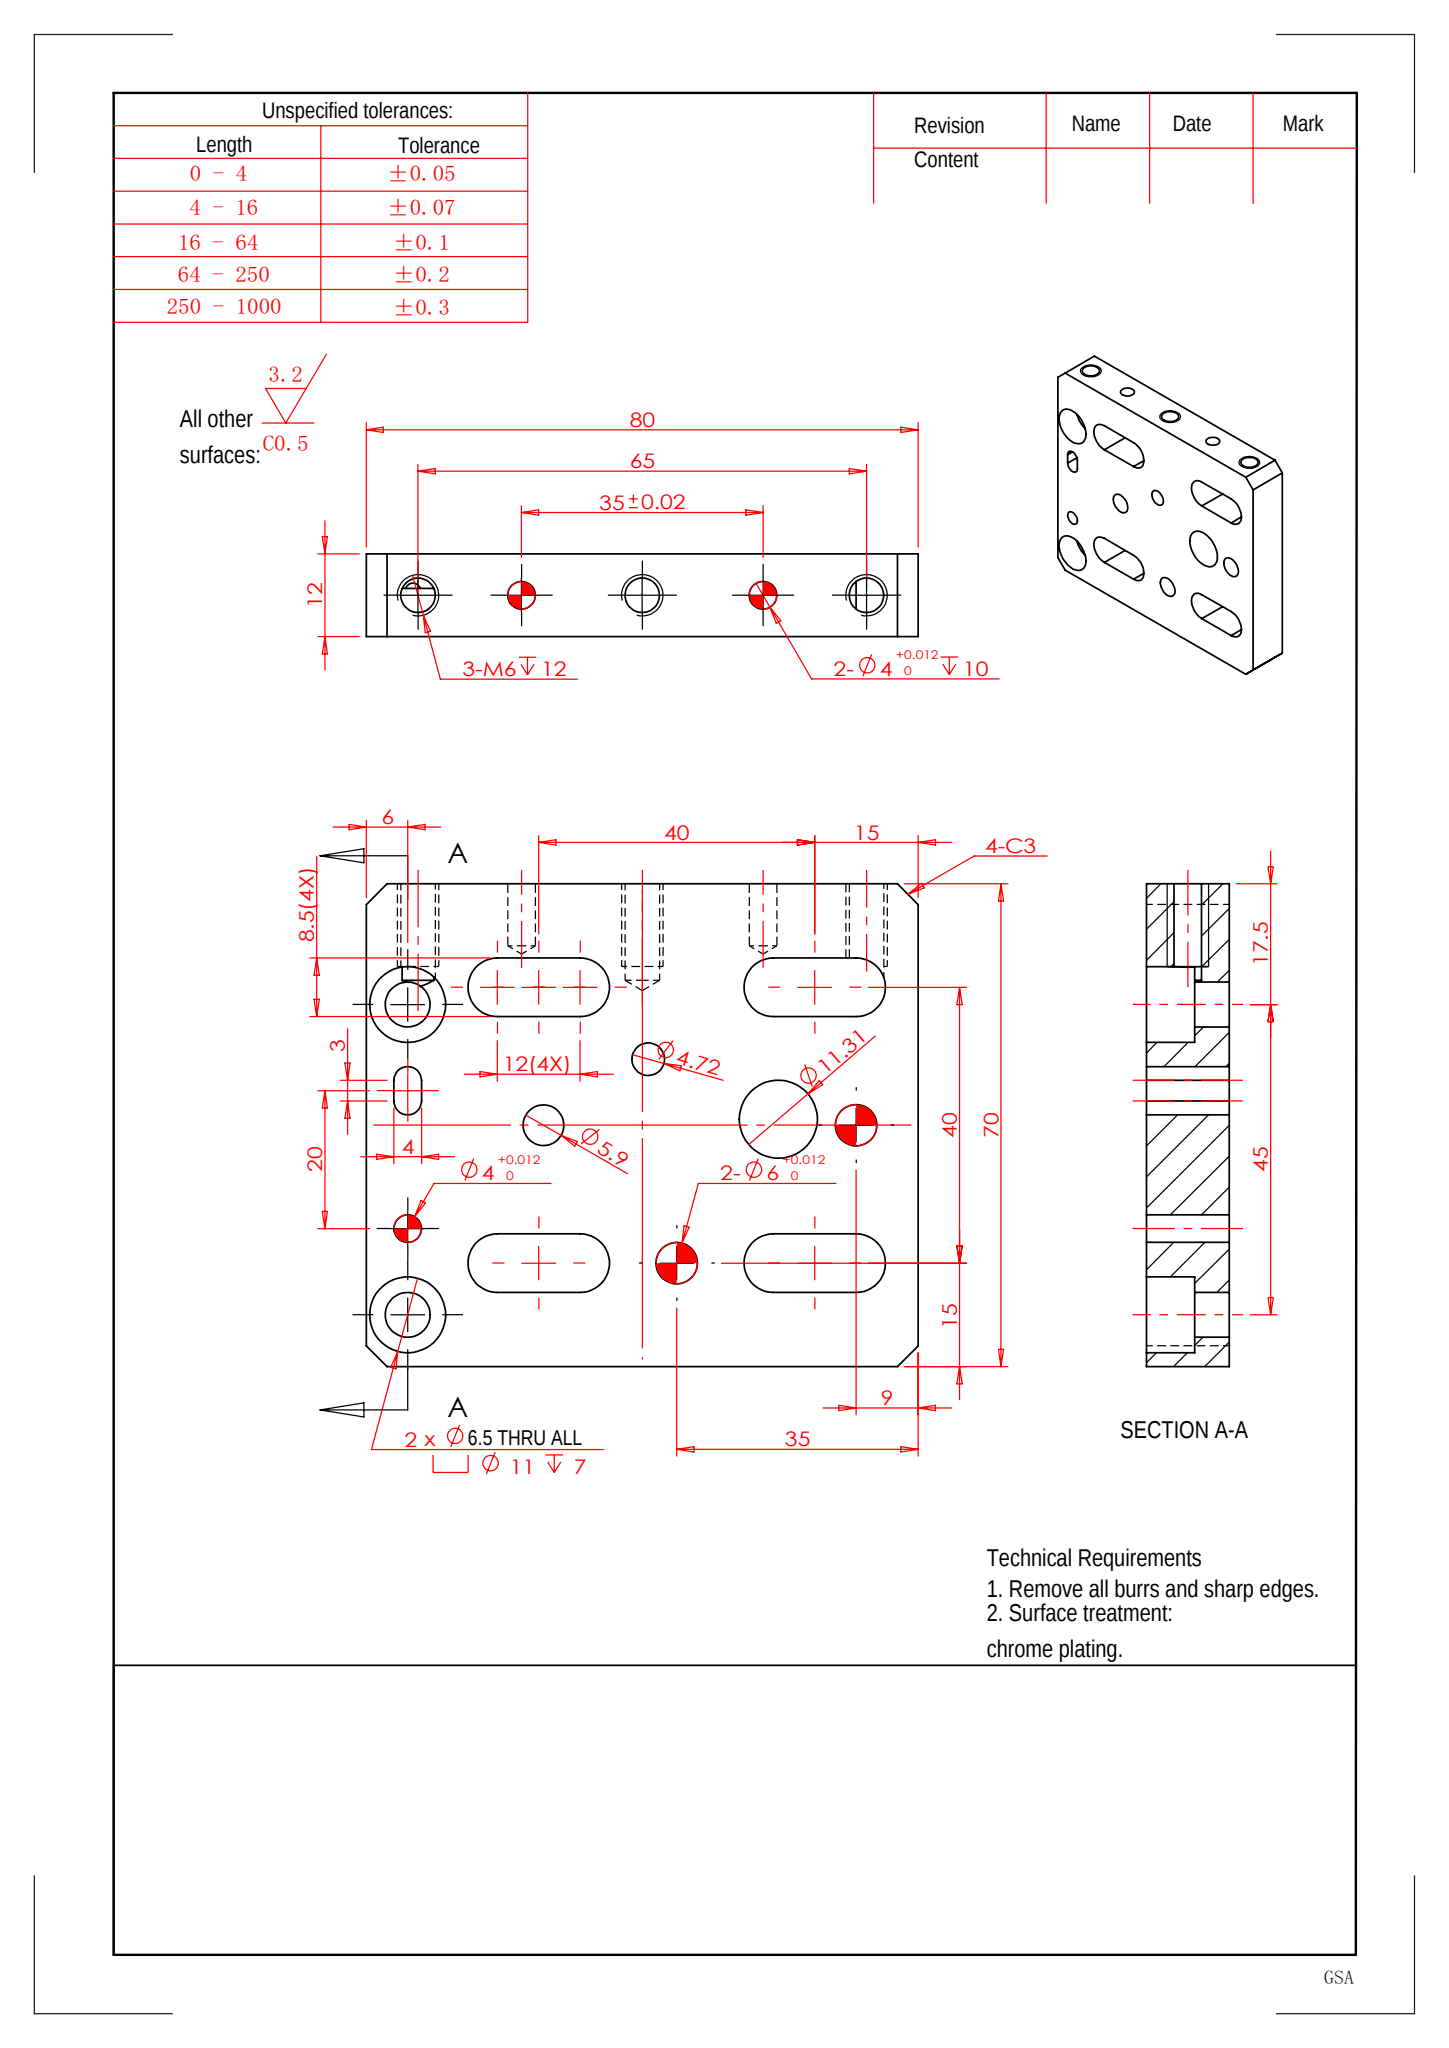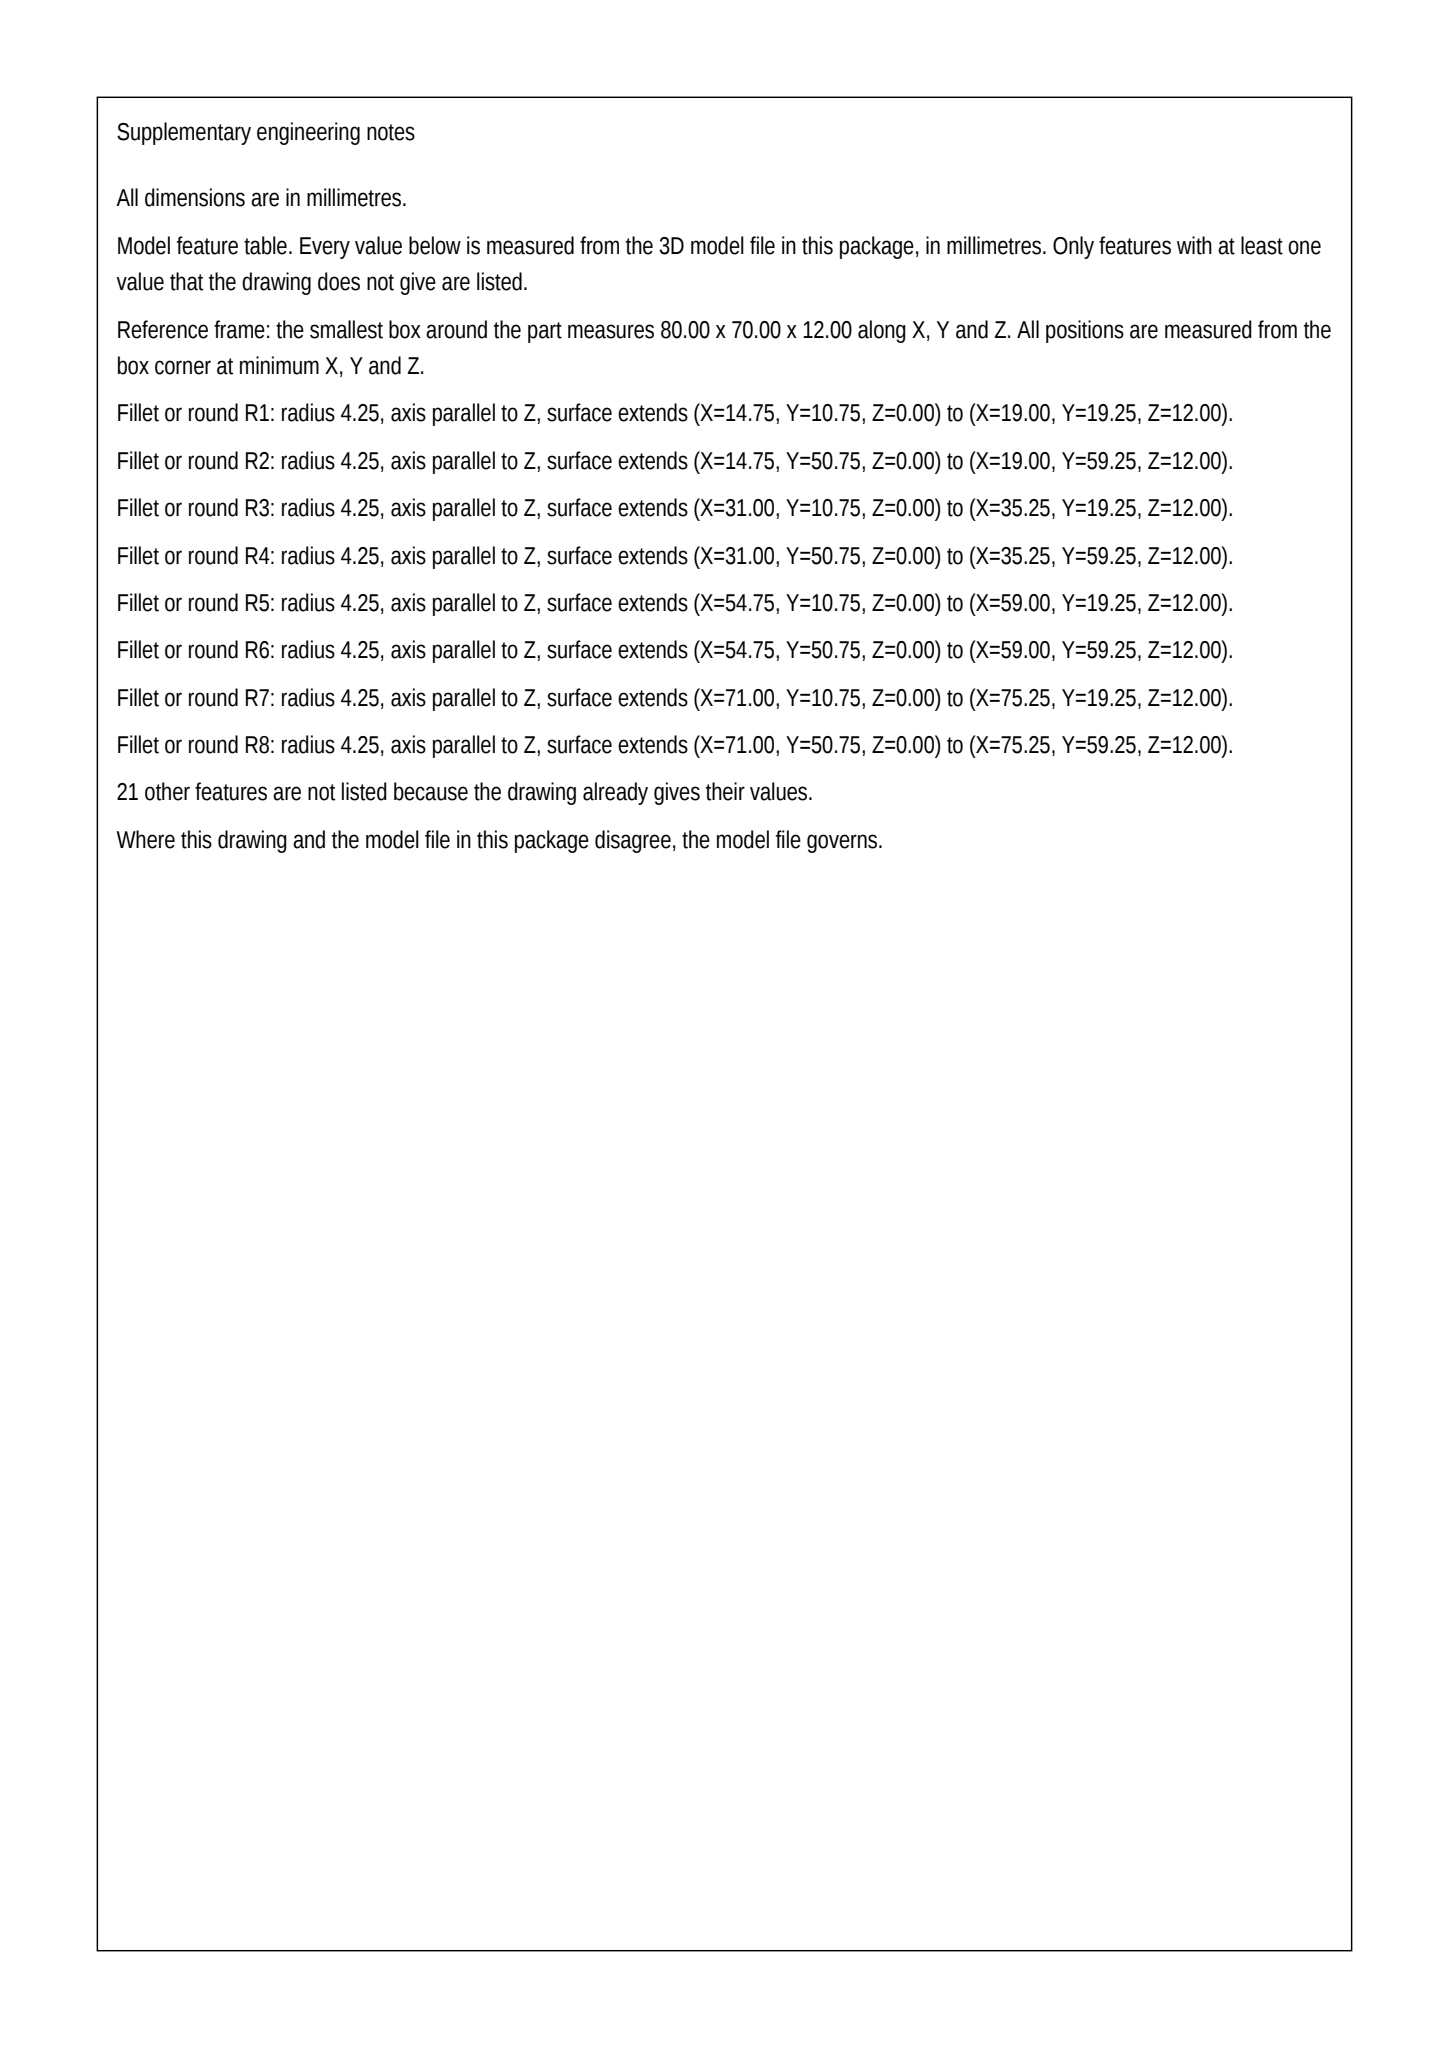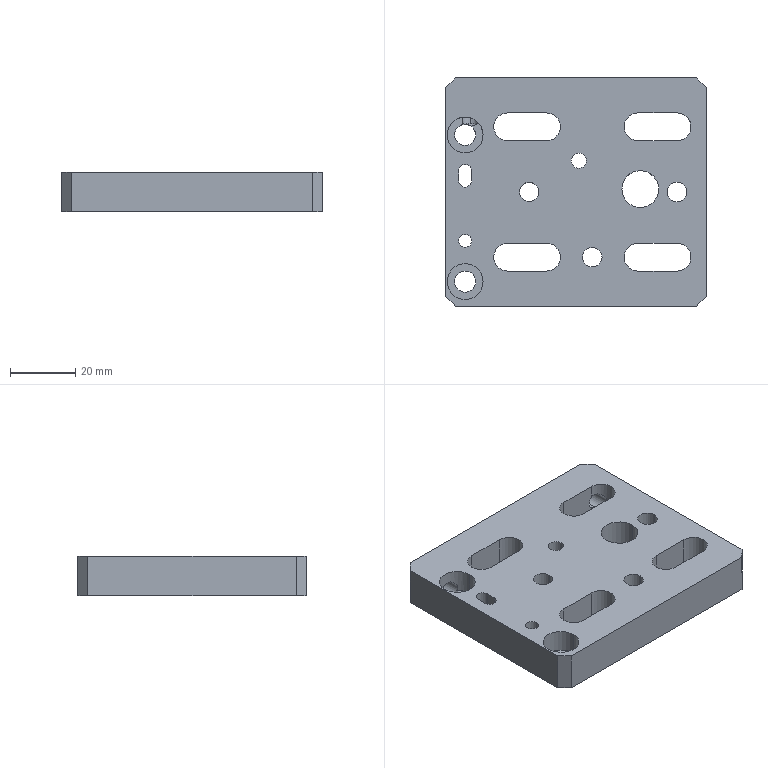Part | SolidWorks | mm | 1 solid | 73 faces | box 80 x 70 x 12 mm | volume 53839 mm3 | cylinder 44 | plane 22 | cone 7 | commonest cylinder face diameters 8.5 x12 4 x8 5 x6 6 x4 11 x4 6.5 x4 11.308 x2 5.905 x2
Drawing notes:
Ø4.72 THRU: 40.9 FROM LEFT EDGE, 44.6 FROM BTM EDGE | from the solid: hole/bore dia 4.72, axis z at [40.9, 44.6], z 0->12 (thru 12 thk)
Ø5.9 THRU: 25.7 FROM LEFT EDGE, 35 FROM BTM EDGE (ON HORIZ CL) | from the solid: hole/bore dia 5.9, axis z at [25.7, 35.0], z 0->12; bbox Y=70 so 35=CL
Ø11.31 THRU: 59.7 FROM LEFT EDGE, 35.9 FROM BTM EDGE | from the solid: hole/bore dia 11.31, axis z at [59.7, 35.9], z 0->12
SEC A-A LEFT SLOT 4 WIDE: THRU, FULL THK 12 (NO STEP) | from the solid: planes x=4.0 & x=8.0, y 38.5-41.5, z 0-12; end arcs R2 z 0-12
Ø4 +0.012/0 THRU: 6 FROM LEFT EDGE, 20 FROM BTM EDGE | from the solid: hole/bore dia 4.0, axis z at [6.0, 20.0], z 0->12
OBROUND SLOT Ø4 CTRS 3: CTR 6 FROM LEFT EDGE, 40 FROM BTM EDGE | from the solid: arcs dia 4 at [6,38.5] & [6,41.5] (ctrs 3 apart, midpt y=40), thru z 0-12
build123d program:
from build123d import *

# Parameters (mm, degrees)
SKETCH1_W                                            = 80
SKETCH1_H                                            = 70
BOSS_EXTRUDE1_DEPTH                                  = 12
CUT_EXTRUDE1_DEPTH                                   = 55.489
M6_TAPPED_HOLE1_D                                    = 5
M6_TAPPED_HOLE1_DEPTH                                = 14
M6_TAPPED_HOLE1_TIP                                  = 1.502
F_4_0_4_DIAMETER_HOLE1_D                             = 4
F_4_0_4_DIAMETER_HOLE1_DEPTH                         = 9
F_4_0_4_DIAMETER_HOLE1_TIP                           = 1.202
HOLE_SIZE_ACCORDING_TO_HEX_SOCKET_HEAD_C_D           = 6.5
HOLE_SIZE_ACCORDING_TO_HEX_SOCKET_HEAD_C_CBORE_D     = 11
HOLE_SIZE_ACCORDING_TO_HEX_SOCKET_HEAD_C_CBORE_DEPTH = 7
F_4_0_4_DIAMETER_HOLE2_D                             = 4
CUT_EXTRUDE3_DEPTH                                   = 55.489
CHAMFER1_SIZE                                        = 3
SKETCH13_R                                           = 3
CUT_EXTRUDE4_DEPTH                                   = 55.489
SKETCH14_R                                           = 5.654
SKETCH14_R_2                                         = 2.952
SKETCH14_R_3                                         = 2.361
CUT_EXTRUDE5_DEPTH                                   = 33


with BuildPart() as part:
    # Sketch1 → Boss-Extrude1 (new body)
    with BuildSketch(Plane.XY):
        Rectangle(SKETCH1_W, SKETCH1_H)
    extrude(amount=BOSS_EXTRUDE1_DEPTH)

    # Sketch2 → Cut-Extrude1 (cut, through all)
    with BuildSketch(Plane(origin=(0, 0, 0), x_dir=(-1, 0, 0), z_dir=(0, 0, -1))):
        with BuildLine():
            Line((21, -24.25), (9, -24.25))
            ThreePointArc((9, -24.25), (4.75, -20), (9, -15.75))
            Line((9, -15.75), (21, -15.75))
            ThreePointArc((21, -15.75), (25.25, -20), (21, -24.25))
        make_face()
        with BuildLine():
            Line((-19, -24.25), (-31, -24.25))
            ThreePointArc((-31, -24.25), (-35.25, -20), (-31, -15.75))
            Line((-31, -15.75), (-19, -15.75))
            ThreePointArc((-19, -15.75), (-14.75, -20), (-19, -24.25))
        make_face()
        with BuildLine():
            Line((21, 15.75), (9, 15.75))
            ThreePointArc((9, 15.75), (4.75, 20), (9, 24.25))
            Line((9, 24.25), (21, 24.25))
            ThreePointArc((21, 24.25), (25.25, 20), (21, 15.75))
        make_face()
        with BuildLine():
            Line((-19, 15.75), (-31, 15.75))
            ThreePointArc((-31, 15.75), (-35.25, 20), (-31, 24.25))
            Line((-31, 24.25), (-19, 24.25))
            ThreePointArc((-19, 24.25), (-14.75, 20), (-19, 15.75))
        make_face()
    extrude(amount=-CUT_EXTRUDE1_DEPTH, mode=Mode.SUBTRACT)

    # M6 Tapped Hole1
    with Locations(Plane(origin=(-32.5, 35, 6), x_dir=(0, 0, 1), z_dir=(0, 1, 0))):
        with Locations((0, 0), (0, 32.5), (0, 65)):
            Hole(M6_TAPPED_HOLE1_D / 2, depth=M6_TAPPED_HOLE1_DEPTH)
            with Locations((0, 0, -(M6_TAPPED_HOLE1_DEPTH + M6_TAPPED_HOLE1_TIP / 2))):  # 118° drill point
                Cone(0, M6_TAPPED_HOLE1_D / 2, M6_TAPPED_HOLE1_TIP, mode=Mode.SUBTRACT)

    # 4.0 _4_ Diameter Hole1
    with Locations(Plane(origin=(-17.5, 35, 6), x_dir=(0, 0, 1), z_dir=(0, 1, 0))):
        with Locations((0, 0), (0, 35)):
            Hole(F_4_0_4_DIAMETER_HOLE1_D / 2, depth=F_4_0_4_DIAMETER_HOLE1_DEPTH)
            with Locations((0, 0, -(F_4_0_4_DIAMETER_HOLE1_DEPTH + F_4_0_4_DIAMETER_HOLE1_TIP / 2))):  # 118° drill point
                Cone(0, F_4_0_4_DIAMETER_HOLE1_D / 2, F_4_0_4_DIAMETER_HOLE1_TIP, mode=Mode.SUBTRACT)

    # Hole Size according to Hex Socket Head C (through all)
    with Locations(Plane.XY.offset(12)):
        with Locations((-34, -27.5), (-34, 17.5)):
            CounterBoreHole(HOLE_SIZE_ACCORDING_TO_HEX_SOCKET_HEAD_C_D / 2, HOLE_SIZE_ACCORDING_TO_HEX_SOCKET_HEAD_C_CBORE_D / 2, HOLE_SIZE_ACCORDING_TO_HEX_SOCKET_HEAD_C_CBORE_DEPTH)

    # 4.0 _4_ Diameter Hole2 (through all)
    with Locations(Plane.XY.offset(12)):
        with Locations((-33.992, -15), (-33.992, 5)):
            Hole(F_4_0_4_DIAMETER_HOLE2_D / 2)

    # Sketch12 → Cut-Extrude3 (cut, through all)
    with BuildSketch(Plane.XY.offset(12)):
        with BuildLine():
            Line((-35.992, 3.5), (-35.992, 6.5))
            ThreePointArc((-35.992, 6.5), (-33.992, 8.5), (-31.992, 6.5))
            Line((-31.992, 6.5), (-31.992, 3.5))
            ThreePointArc((-31.992, 3.5), (-33.992, 1.5), (-35.992, 3.5))
        make_face()
    extrude(amount=-CUT_EXTRUDE3_DEPTH, mode=Mode.SUBTRACT)

    # Chamfer1
    chamfer1_edges = [part.edges().sort_by_distance(p)[0] for p in [
        (40, -35, 6),
        (-40, -35, 6),
        (-40, 35, 6),
        (40, 35, 6),
    ]]
    chamfer(chamfer1_edges, length=CHAMFER1_SIZE)

    # Sketch13 → Cut-Extrude4 (cut, through all)
    with BuildSketch(Plane(origin=(0, 0, 0), x_dir=(-1, 0, 0), z_dir=(0, 0, -1))):
        with Locations((-31, 0)):
            Circle(SKETCH13_R)
        with Locations((-5, -20)):
            Circle(SKETCH13_R)
    extrude(amount=-CUT_EXTRUDE4_DEPTH, mode=Mode.SUBTRACT)

    # Sketch14 → Cut-Extrude5 (cut)
    with BuildSketch(Plane(origin=(0, 0, 0), x_dir=(-1, 0, 0), z_dir=(0, 0, -1))):
        with Locations((-19.729, 0.8704)):
            Circle(SKETCH14_R)
        with Locations((14.313, 0)):
            Circle(SKETCH14_R_2)
        with Locations((-0.8704, 9.574)):
            Circle(SKETCH14_R_3)
    extrude(amount=-CUT_EXTRUDE5_DEPTH, mode=Mode.SUBTRACT)


solid = part.part